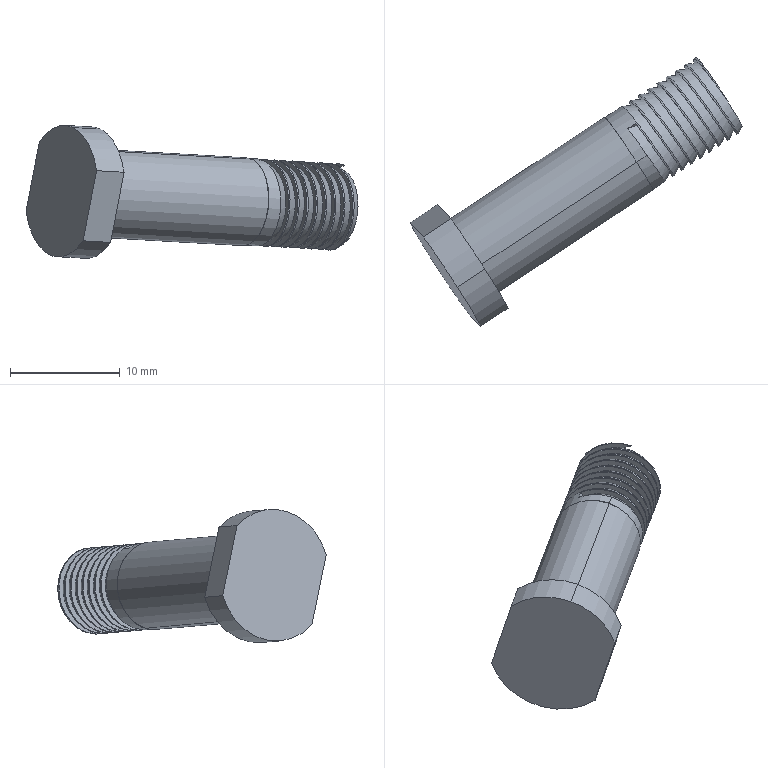Component | SolidWorks | DoorFisheyeShaftPin-1 | 1 solid | 32 faces | volume 1616 mm3 | cylinder 23 | plane 7 | spline 2 | commonest cylinder face diameters 7.9 x18 12 x3 8 x2